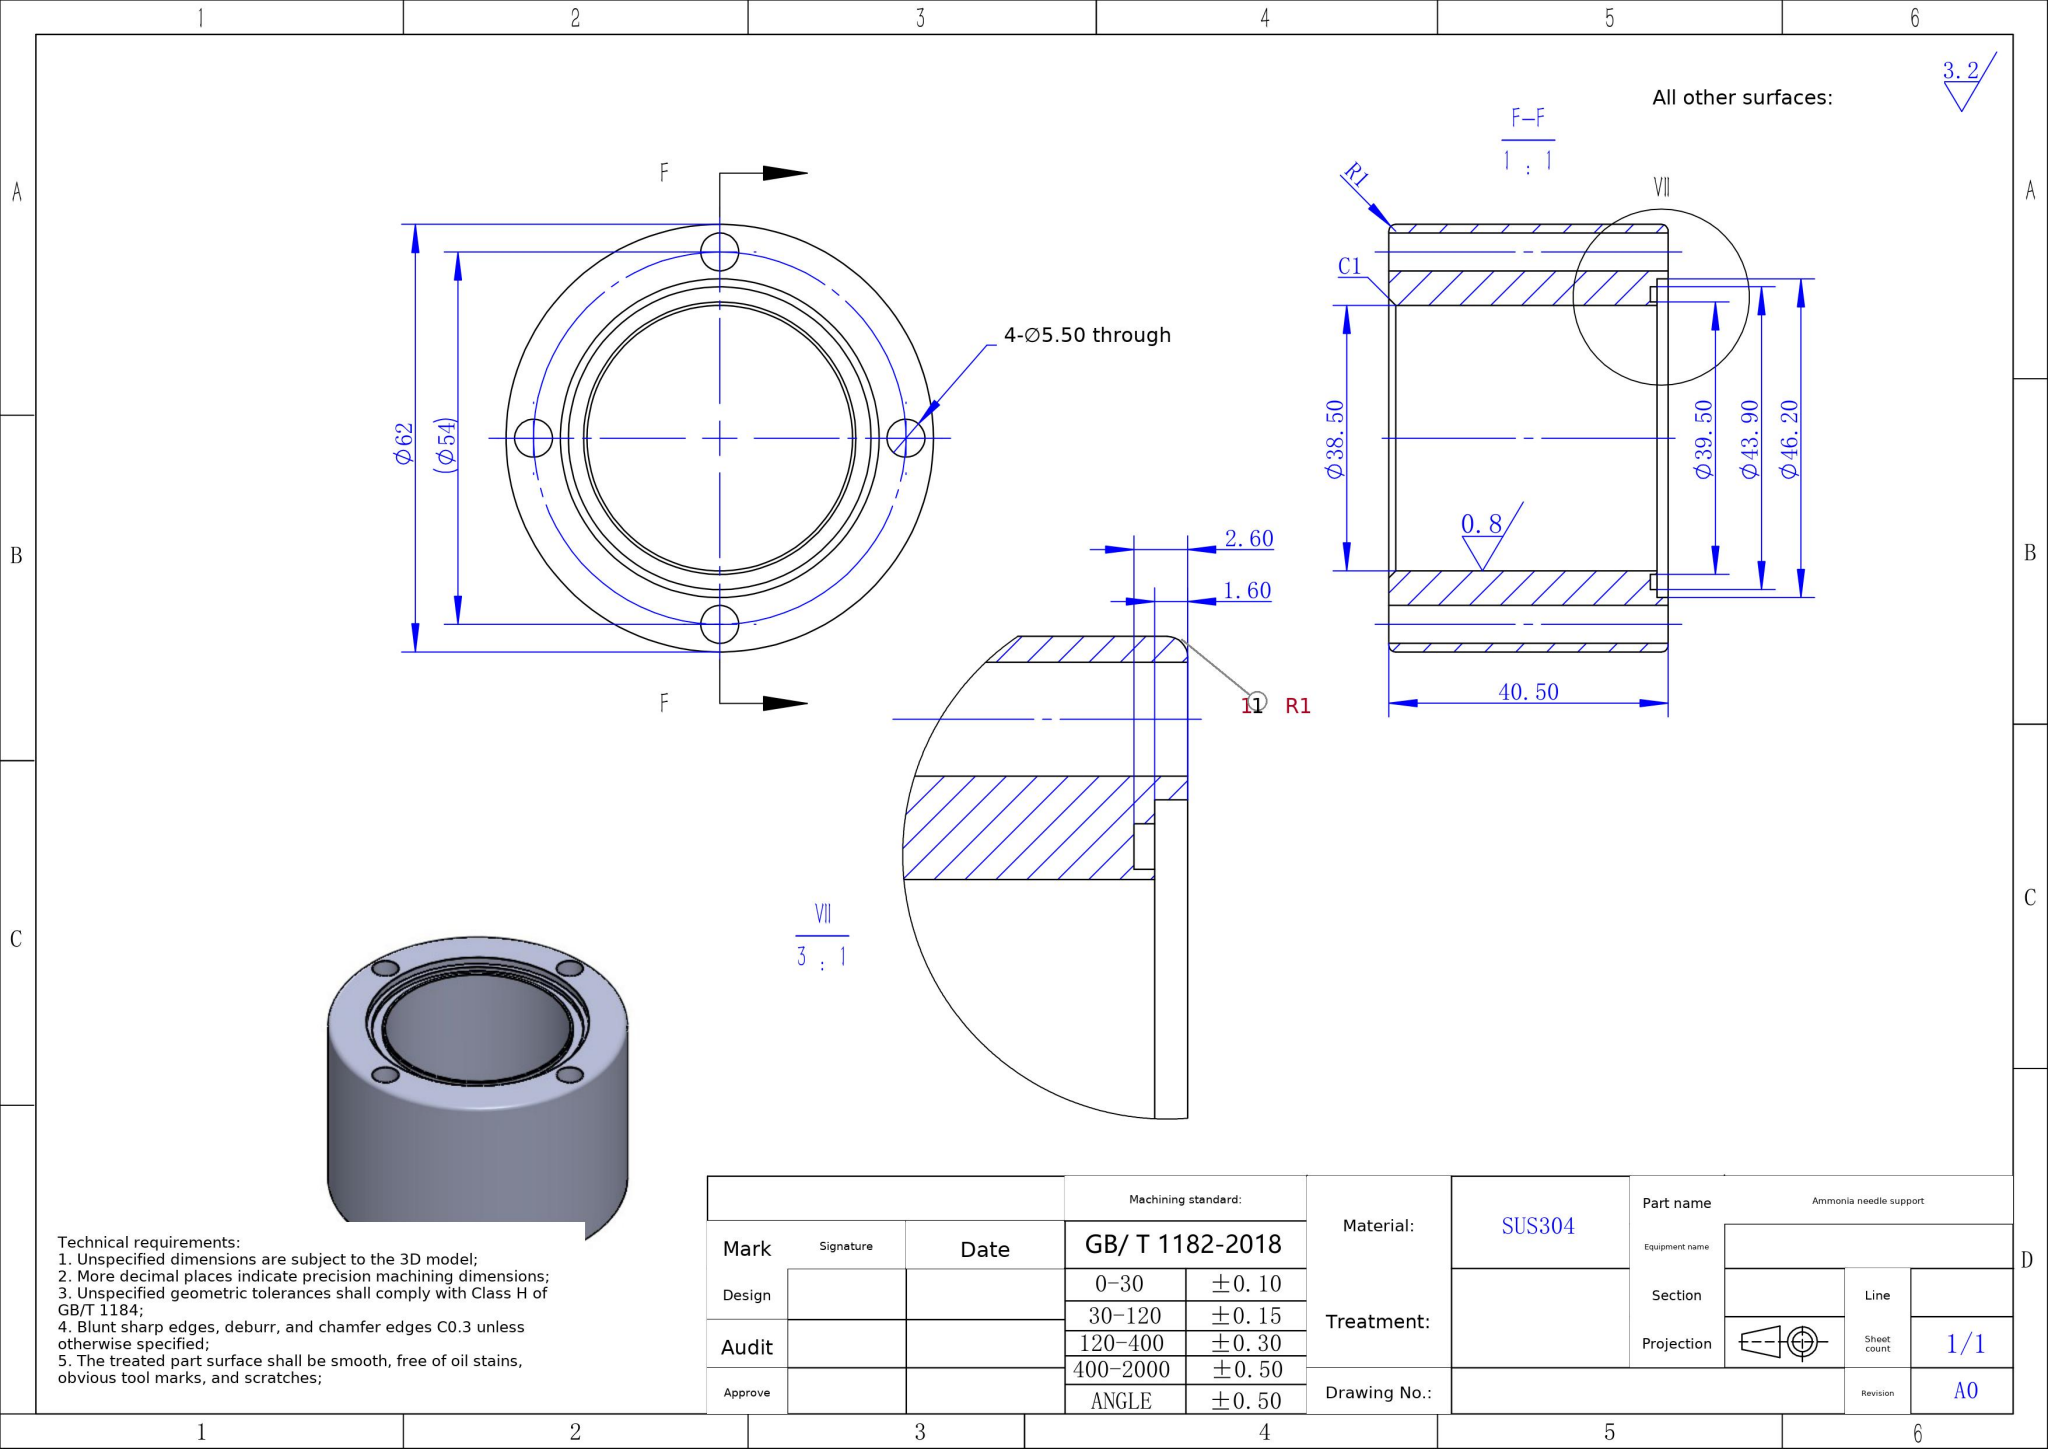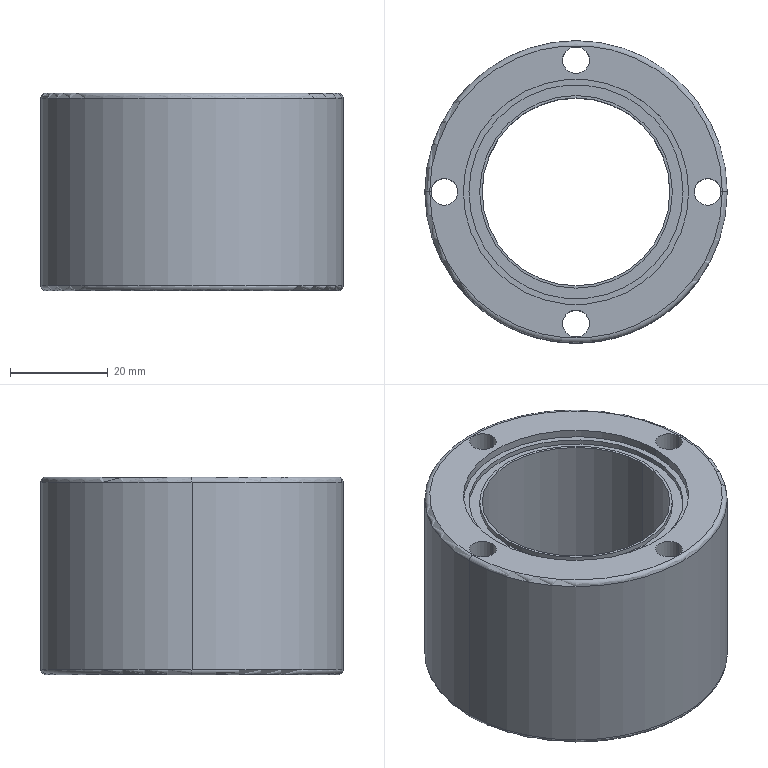Part | SolidWorks | mm | material SUS304 | 1 solid | 29 faces | box 62 x 62 x 40.5 mm | volume 70023 mm3 | cylinder 18 | plane 5 | torus 4 | cone 2 | commonest cylinder face diameters 5.5 x8 39.5 x2 43.9 x2 46.2 x2 62 x2 38.5 x2
build123d program:
from build123d import *

# Parameters (mm, degrees)
SKETCH1_R           = 31
BOSS_EXTRUDE1_DEPTH = 40.5
SKETCH2_R           = 19.25
CUT_EXTRUDE1_DEPTH  = 40.5
SKETCH3_R           = 2.75
CUT_EXTRUDE2_DEPTH  = 60.685
FILLET1_R           = 1
CHAMFER1_SIZE       = 1
SKETCH4_R           = 23.1
CUT_EXTRUDE3_DEPTH  = 1.6
SKETCH5_R           = 21.95
CUT_EXTRUDE4_DEPTH  = 1
BOSS_EXTRUDE2_START = 1
SKETCH6_R           = 19.75
SKETCH6_R_2         = 19.25
BOSS_EXTRUDE2_DEPTH = 1


with BuildPart() as part:
    # Sketch1 → Boss-Extrude1 (new body)
    with BuildSketch(Plane.XY):
        Circle(SKETCH1_R)
    extrude(amount=BOSS_EXTRUDE1_DEPTH)

    # Sketch2 → Cut-Extrude1 (cut)
    with BuildSketch(Plane.XY.offset(40.5)):
        Circle(SKETCH2_R)
    extrude(amount=-CUT_EXTRUDE1_DEPTH, mode=Mode.SUBTRACT)

    # Sketch3 → Cut-Extrude2 (cut, through all)
    with BuildSketch(Plane.XY.offset(40.5)):
        with Locations((0, 27)):
            Circle(SKETCH3_R)
        with Locations((27, 0)):
            Circle(SKETCH3_R)
        with Locations((0, -27)):
            Circle(SKETCH3_R)
        with Locations((-27, 0)):
            Circle(SKETCH3_R)
    extrude(amount=-CUT_EXTRUDE2_DEPTH, mode=Mode.SUBTRACT)

    # Fillet1
    fillet1_edges = [part.edges().sort_by_distance(p)[0] for p in [
        (-31, 0, 0),
        (-31, 0, 40.5),
    ]]
    fillet(fillet1_edges, radius=FILLET1_R)

    # Chamfer1
    chamfer1_edges = [part.edges().sort_by_distance(p)[0] for p in [
        (-19.25, 0, 0),
    ]]
    chamfer(chamfer1_edges, length=CHAMFER1_SIZE)

    # Sketch4 → Cut-Extrude3 (cut)
    with BuildSketch(Plane.XY.offset(40.5)):
        Circle(SKETCH4_R)
    extrude(amount=-CUT_EXTRUDE3_DEPTH, mode=Mode.SUBTRACT)

    # Sketch5 → Cut-Extrude4 (cut)
    with BuildSketch(Plane.XY.offset(38.9)):
        Circle(SKETCH5_R)
    extrude(amount=-CUT_EXTRUDE4_DEPTH, mode=Mode.SUBTRACT)

    # Sketch6 → Boss-Extrude2 (add)
    with BuildSketch(Plane.XY.offset(37.9).offset(BOSS_EXTRUDE2_START)):
        Circle(SKETCH6_R)
        Circle(SKETCH6_R_2, mode=Mode.SUBTRACT)
    extrude(amount=-BOSS_EXTRUDE2_DEPTH)


solid = part.part
STEP:
#1=CARTESIAN_POINT('',(19.75,0.,38.9));
#2=VERTEX_POINT('',#1);
#3=CARTESIAN_POINT('',(-19.75,0.,38.9));
#4=VERTEX_POINT('',#3);
#5=CARTESIAN_POINT('',(0.,0.,38.9));
#6=DIRECTION('',(0.,0.,1.));
#7=DIRECTION('',(1.,0.,0.));
#8=AXIS2_PLACEMENT_3D('',#5,#6,#7);
#9=CIRCLE('',#8,19.75);
#10=EDGE_CURVE('',#2,#4,#9,.T.);
#11=ORIENTED_EDGE('',*,*,#10,.F.);
#12=CARTESIAN_POINT('',(19.75,0.,37.9));
#13=VERTEX_POINT('',#12);
#14=CARTESIAN_POINT('',(19.75,0.,38.9));
#15=DIRECTION('',(0.,0.,-1.));
#16=VECTOR('',#15,1000.);
#17=LINE('',#14,#16);
#18=EDGE_CURVE('',#2,#13,#17,.T.);
#19=ORIENTED_EDGE('',*,*,#18,.T.);
#20=CARTESIAN_POINT('',(-19.75,0.,37.9));
#21=VERTEX_POINT('',#20);
#22=CARTESIAN_POINT('',(0.,0.,37.9));
#23=DIRECTION('',(0.,0.,1.));
#24=DIRECTION('',(1.,0.,0.));
#25=AXIS2_PLACEMENT_3D('',#22,#23,#24);
#26=CIRCLE('',#25,19.75);
#27=EDGE_CURVE('',#13,#21,#26,.T.);
#28=ORIENTED_EDGE('',*,*,#27,.T.);
#29=CARTESIAN_POINT('',(-19.75,0.,38.9));
#30=DIRECTION('',(0.,0.,-1.));
#31=VECTOR('',#30,1000.);
#32=LINE('',#29,#31);
#33=EDGE_CURVE('',#4,#21,#32,.T.);
#34=ORIENTED_EDGE('',*,*,#33,.F.);
#35=EDGE_LOOP('',(#11,#19,#28,#34));
#36=FACE_OUTER_BOUND('',#35,.T.);
#37=CARTESIAN_POINT('',(0.,0.,38.9));
#38=DIRECTION('',(0.,0.,-1.));
#39=DIRECTION('',(-1.,0.,0.));
#40=AXIS2_PLACEMENT_3D('',#37,#38,#39);
#41=CYLINDRICAL_SURFACE('',#40,19.75);
#42=ADVANCED_FACE('',(#36),#41,.T.);
#43=CARTESIAN_POINT('',(-21.95,0.,37.9));
#44=VERTEX_POINT('',#43);
#45=CARTESIAN_POINT('',(21.95,0.,37.9));
#46=VERTEX_POINT('',#45);
#47=CARTESIAN_POINT('',(0.,0.,37.9));
#48=DIRECTION('',(0.,0.,1.));
#49=DIRECTION('',(1.,0.,0.));
#50=AXIS2_PLACEMENT_3D('',#47,#48,#49);
#51=CIRCLE('',#50,21.95);
#52=EDGE_CURVE('',#44,#46,#51,.T.);
#53=ORIENTED_EDGE('',*,*,#52,.F.);
#54=CARTESIAN_POINT('',(-21.95,0.,38.9));
#55=VERTEX_POINT('',#54);
#56=CARTESIAN_POINT('',(-21.95,0.,37.9));
#57=DIRECTION('',(0.,0.,1.));
#58=VECTOR('',#57,1000.);
#59=LINE('',#56,#58);
#60=EDGE_CURVE('',#44,#55,#59,.T.);
#61=ORIENTED_EDGE('',*,*,#60,.T.);
#62=CARTESIAN_POINT('',(21.95,0.,38.9));
#63=VERTEX_POINT('',#62);
#64=CARTESIAN_POINT('',(0.,0.,38.9));
#65=DIRECTION('',(0.,0.,1.));
#66=DIRECTION('',(1.,0.,0.));
#67=AXIS2_PLACEMENT_3D('',#64,#65,#66);
#68=CIRCLE('',#67,21.95);
#69=EDGE_CURVE('',#55,#63,#68,.T.);
#70=ORIENTED_EDGE('',*,*,#69,.T.);
#71=CARTESIAN_POINT('',(21.95,0.,37.9));
#72=DIRECTION('',(0.,0.,1.));
#73=VECTOR('',#72,1000.);
#74=LINE('',#71,#73);
#75=EDGE_CURVE('',#46,#63,#74,.T.);
#76=ORIENTED_EDGE('',*,*,#75,.F.);
#77=EDGE_LOOP('',(#53,#61,#70,#76));
#78=FACE_OUTER_BOUND('',#77,.T.);
#79=CARTESIAN_POINT('',(0.,0.,37.9));
#80=DIRECTION('',(0.,0.,1.));
#81=DIRECTION('',(1.,0.,0.));
#82=AXIS2_PLACEMENT_3D('',#79,#80,#81);
#83=CYLINDRICAL_SURFACE('',#82,21.95);
#84=ADVANCED_FACE('',(#78),#83,.F.);
#85=CARTESIAN_POINT('',(-23.1,0.,38.9));
#86=VERTEX_POINT('',#85);
#87=CARTESIAN_POINT('',(23.1,0.,38.9));
#88=VERTEX_POINT('',#87);
#89=CARTESIAN_POINT('',(0.,0.,38.9));
#90=DIRECTION('',(0.,0.,1.));
#91=DIRECTION('',(1.,0.,0.));
#92=AXIS2_PLACEMENT_3D('',#89,#90,#91);
#93=CIRCLE('',#92,23.1);
#94=EDGE_CURVE('',#86,#88,#93,.T.);
#95=ORIENTED_EDGE('',*,*,#94,.F.);
#96=CARTESIAN_POINT('',(-23.1,0.,40.5));
#97=VERTEX_POINT('',#96);
#98=CARTESIAN_POINT('',(-23.1,0.,38.9));
#99=DIRECTION('',(0.,0.,1.));
#100=VECTOR('',#99,1000.);
#101=LINE('',#98,#100);
#102=EDGE_CURVE('',#86,#97,#101,.T.);
#103=ORIENTED_EDGE('',*,*,#102,.T.);
#104=CARTESIAN_POINT('',(23.1,0.,40.5));
#105=VERTEX_POINT('',#104);
#106=CARTESIAN_POINT('',(0.,0.,40.5));
#107=DIRECTION('',(0.,0.,1.));
#108=DIRECTION('',(1.,0.,0.));
#109=AXIS2_PLACEMENT_3D('',#106,#107,#108);
#110=CIRCLE('',#109,23.1);
#111=EDGE_CURVE('',#97,#105,#110,.T.);
#112=ORIENTED_EDGE('',*,*,#111,.T.);
#113=CARTESIAN_POINT('',(23.1,0.,38.9));
#114=DIRECTION('',(0.,0.,1.));
#115=VECTOR('',#114,1000.);
#116=LINE('',#113,#115);
#117=EDGE_CURVE('',#88,#105,#116,.T.);
#118=ORIENTED_EDGE('',*,*,#117,.F.);
#119=EDGE_LOOP('',(#95,#103,#112,#118));
#120=FACE_OUTER_BOUND('',#119,.T.);
#121=CARTESIAN_POINT('',(0.,0.,38.9));
#122=DIRECTION('',(0.,0.,1.));
#123=DIRECTION('',(1.,0.,0.));
#124=AXIS2_PLACEMENT_3D('',#121,#122,#123);
#125=CYLINDRICAL_SURFACE('',#124,23.1);
#126=ADVANCED_FACE('',(#120),#125,.F.);
#127=CARTESIAN_POINT('',(19.25,0.,1.));
#128=VERTEX_POINT('',#127);
#129=CARTESIAN_POINT('',(-19.25,0.,1.));
#130=VERTEX_POINT('',#129);
#131=CARTESIAN_POINT('',(0.,0.,1.));
#132=DIRECTION('',(0.,0.,-1.));
#133=DIRECTION('',(1.,0.,0.));
#134=AXIS2_PLACEMENT_3D('',#131,#132,#133);
#135=CIRCLE('',#134,19.25);
#136=EDGE_CURVE('',#128,#130,#135,.T.);
#137=ORIENTED_EDGE('',*,*,#136,.F.);
#138=CARTESIAN_POINT('',(20.25,0.,0.));
#139=VERTEX_POINT('',#138);
#140=CARTESIAN_POINT('',(20.25,0.,0.));
#141=DIRECTION('',(0.7071,0.,-0.7071));
#142=VECTOR('',#141,1000.);
#143=LINE('',#140,#142);
#144=EDGE_CURVE('',#128,#139,#143,.T.);
#145=ORIENTED_EDGE('',*,*,#144,.T.);
#146=CARTESIAN_POINT('',(-20.25,0.,0.));
#147=VERTEX_POINT('',#146);
#148=CARTESIAN_POINT('',(0.,0.,0.));
#149=DIRECTION('',(0.,0.,1.));
#150=DIRECTION('',(1.,0.,0.));
#151=AXIS2_PLACEMENT_3D('',#148,#149,#150);
#152=CIRCLE('',#151,20.25);
#153=EDGE_CURVE('',#147,#139,#152,.T.);
#154=ORIENTED_EDGE('',*,*,#153,.F.);
#155=CARTESIAN_POINT('',(-20.25,0.,0.));
#156=DIRECTION('',(-0.7071,0.,-0.7071));
#157=VECTOR('',#156,1000.);
#158=LINE('',#155,#157);
#159=EDGE_CURVE('',#130,#147,#158,.T.);
#160=ORIENTED_EDGE('',*,*,#159,.F.);
#161=EDGE_LOOP('',(#137,#145,#154,#160));
#162=FACE_OUTER_BOUND('',#161,.T.);
#163=CARTESIAN_POINT('',(0.,0.,0.));
#164=DIRECTION('',(0.,0.,-1.));
#165=DIRECTION('',(-1.,0.,0.));
#166=AXIS2_PLACEMENT_3D('',#163,#164,#165);
#167=CONICAL_SURFACE('',#166,20.25,0.7854);
#168=ADVANCED_FACE('',(#162),#167,.F.);
#169=CARTESIAN_POINT('',(-31.,0.,39.5));
#170=VERTEX_POINT('',#169);
#171=CARTESIAN_POINT('',(31.,0.,39.5));
#172=VERTEX_POINT('',#171);
#173=CARTESIAN_POINT('',(0.,0.,39.5));
#174=DIRECTION('',(0.,0.,-1.));
#175=DIRECTION('',(1.,0.,0.));
#176=AXIS2_PLACEMENT_3D('',#173,#174,#175);
#177=CIRCLE('',#176,31.);
#178=EDGE_CURVE('',#170,#172,#177,.T.);
#179=ORIENTED_EDGE('',*,*,#178,.F.);
#180=CARTESIAN_POINT('',(-30.,0.,40.5));
#181=VERTEX_POINT('',#180);
#182=CARTESIAN_POINT('',(-30.,0.,39.5));
#183=DIRECTION('',(0.,1.,0.));
#184=DIRECTION('',(-1.,0.,0.));
#185=AXIS2_PLACEMENT_3D('',#182,#183,#184);
#186=CIRCLE('',#185,1.);
#187=EDGE_CURVE('',#170,#181,#186,.T.);
#188=ORIENTED_EDGE('',*,*,#187,.T.);
#189=CARTESIAN_POINT('',(30.,0.,40.5));
#190=VERTEX_POINT('',#189);
#191=CARTESIAN_POINT('',(0.,0.,40.5));
#192=DIRECTION('',(0.,0.,1.));
#193=DIRECTION('',(1.,0.,0.));
#194=AXIS2_PLACEMENT_3D('',#191,#192,#193);
#195=CIRCLE('',#194,30.);
#196=EDGE_CURVE('',#190,#181,#195,.T.);
#197=ORIENTED_EDGE('',*,*,#196,.F.);
#198=CARTESIAN_POINT('',(30.,0.,39.5));
#199=DIRECTION('',(0.,-1.,0.));
#200=DIRECTION('',(0.,0.,-1.));
#201=AXIS2_PLACEMENT_3D('',#198,#199,#200);
#202=CIRCLE('',#201,1.);
#203=EDGE_CURVE('',#172,#190,#202,.T.);
#204=ORIENTED_EDGE('',*,*,#203,.F.);
#205=EDGE_LOOP('',(#179,#188,#197,#204));
#206=FACE_OUTER_BOUND('',#205,.T.);
#207=CARTESIAN_POINT('',(0.,0.,39.5));
#208=DIRECTION('',(0.,0.,1.));
#209=DIRECTION('',(1.,0.,0.));
#210=AXIS2_PLACEMENT_3D('',#207,#208,#209);
#211=TOROIDAL_SURFACE('',#210,30.,1.);
#212=ADVANCED_FACE('',(#206),#211,.T.);
#213=CARTESIAN_POINT('',(-30.,0.,0.));
#214=VERTEX_POINT('',#213);
#215=CARTESIAN_POINT('',(30.,0.,0.));
#216=VERTEX_POINT('',#215);
#217=CARTESIAN_POINT('',(0.,0.,0.));
#218=DIRECTION('',(0.,0.,-1.));
#219=DIRECTION('',(1.,0.,0.));
#220=AXIS2_PLACEMENT_3D('',#217,#218,#219);
#221=CIRCLE('',#220,30.);
#222=EDGE_CURVE('',#214,#216,#221,.T.);
#223=ORIENTED_EDGE('',*,*,#222,.F.);
#224=CARTESIAN_POINT('',(-31.,0.,1.));
#225=VERTEX_POINT('',#224);
#226=CARTESIAN_POINT('',(-30.,0.,1.));
#227=DIRECTION('',(0.,1.,0.));
#228=DIRECTION('',(-1.,0.,0.));
#229=AXIS2_PLACEMENT_3D('',#226,#227,#228);
#230=CIRCLE('',#229,1.);
#231=EDGE_CURVE('',#214,#225,#230,.T.);
#232=ORIENTED_EDGE('',*,*,#231,.T.);
#233=CARTESIAN_POINT('',(31.,0.,1.));
#234=VERTEX_POINT('',#233);
#235=CARTESIAN_POINT('',(0.,0.,1.));
#236=DIRECTION('',(0.,0.,1.));
#237=DIRECTION('',(1.,0.,0.));
#238=AXIS2_PLACEMENT_3D('',#235,#236,#237);
#239=CIRCLE('',#238,31.);
#240=EDGE_CURVE('',#234,#225,#239,.T.);
#241=ORIENTED_EDGE('',*,*,#240,.F.);
#242=CARTESIAN_POINT('',(30.,0.,1.));
#243=DIRECTION('',(0.,-1.,0.));
#244=DIRECTION('',(0.,0.,-1.));
#245=AXIS2_PLACEMENT_3D('',#242,#243,#244);
#246=CIRCLE('',#245,1.);
#247=EDGE_CURVE('',#216,#234,#246,.T.);
#248=ORIENTED_EDGE('',*,*,#247,.F.);
#249=EDGE_LOOP('',(#223,#232,#241,#248));
#250=FACE_OUTER_BOUND('',#249,.T.);
#251=CARTESIAN_POINT('',(0.,0.,1.));
#252=DIRECTION('',(0.,0.,1.));
#253=DIRECTION('',(1.,0.,0.));
#254=AXIS2_PLACEMENT_3D('',#251,#252,#253);
#255=TOROIDAL_SURFACE('',#254,30.,1.);
#256=ADVANCED_FACE('',(#250),#255,.T.);
#257=CARTESIAN_POINT('',(-2.75,27.,0.));
#258=VERTEX_POINT('',#257);
#259=CARTESIAN_POINT('',(2.75,27.,0.));
#260=VERTEX_POINT('',#259);
#261=CARTESIAN_POINT('',(0.,27.,0.));
#262=DIRECTION('',(0.,0.,1.));
#263=DIRECTION('',(1.,0.,0.));
#264=AXIS2_PLACEMENT_3D('',#261,#262,#263);
#265=CIRCLE('',#264,2.75);
#266=EDGE_CURVE('',#258,#260,#265,.T.);
#267=ORIENTED_EDGE('',*,*,#266,.F.);
#268=CARTESIAN_POINT('',(-2.75,27.,40.5));
#269=VERTEX_POINT('',#268);
#270=CARTESIAN_POINT('',(-2.75,27.,0.));
#271=DIRECTION('',(0.,0.,1.));
#272=VECTOR('',#271,1000.);
#273=LINE('',#270,#272);
#274=EDGE_CURVE('',#258,#269,#273,.T.);
#275=ORIENTED_EDGE('',*,*,#274,.T.);
#276=CARTESIAN_POINT('',(2.75,27.,40.5));
#277=VERTEX_POINT('',#276);
#278=CARTESIAN_POINT('',(0.,27.,40.5));
#279=DIRECTION('',(0.,0.,1.));
#280=DIRECTION('',(1.,0.,0.));
#281=AXIS2_PLACEMENT_3D('',#278,#279,#280);
#282=CIRCLE('',#281,2.75);
#283=EDGE_CURVE('',#269,#277,#282,.T.);
#284=ORIENTED_EDGE('',*,*,#283,.T.);
#285=CARTESIAN_POINT('',(2.75,27.,0.));
#286=DIRECTION('',(0.,0.,1.));
#287=VECTOR('',#286,1000.);
#288=LINE('',#285,#287);
#289=EDGE_CURVE('',#260,#277,#288,.T.);
#290=ORIENTED_EDGE('',*,*,#289,.F.);
#291=EDGE_LOOP('',(#267,#275,#284,#290));
#292=FACE_OUTER_BOUND('',#291,.T.);
#293=CARTESIAN_POINT('',(0.,27.,0.));
#294=DIRECTION('',(0.,0.,1.));
#295=DIRECTION('',(1.,0.,0.));
#296=AXIS2_PLACEMENT_3D('',#293,#294,#295);
#297=CYLINDRICAL_SURFACE('',#296,2.75);
#298=ADVANCED_FACE('',(#292),#297,.F.);
#299=CARTESIAN_POINT('',(24.25,-0.,0.));
#300=VERTEX_POINT('',#299);
#301=CARTESIAN_POINT('',(29.75,-0.,0.));
#302=VERTEX_POINT('',#301);
#303=CARTESIAN_POINT('',(27.,-0.,0.));
#304=DIRECTION('',(0.,0.,1.));
#305=DIRECTION('',(1.,0.,0.));
#306=AXIS2_PLACEMENT_3D('',#303,#304,#305);
#307=CIRCLE('',#306,2.75);
#308=EDGE_CURVE('',#300,#302,#307,.T.);
#309=ORIENTED_EDGE('',*,*,#308,.F.);
#310=CARTESIAN_POINT('',(24.25,-0.,40.5));
#311=VERTEX_POINT('',#310);
#312=CARTESIAN_POINT('',(24.25,-0.,0.));
#313=DIRECTION('',(0.,0.,1.));
#314=VECTOR('',#313,1000.);
#315=LINE('',#312,#314);
#316=EDGE_CURVE('',#300,#311,#315,.T.);
#317=ORIENTED_EDGE('',*,*,#316,.T.);
#318=CARTESIAN_POINT('',(29.75,-0.,40.5));
#319=VERTEX_POINT('',#318);
#320=CARTESIAN_POINT('',(27.,-0.,40.5));
#321=DIRECTION('',(0.,0.,1.));
#322=DIRECTION('',(1.,0.,0.));
#323=AXIS2_PLACEMENT_3D('',#320,#321,#322);
#324=CIRCLE('',#323,2.75);
#325=EDGE_CURVE('',#311,#319,#324,.T.);
#326=ORIENTED_EDGE('',*,*,#325,.T.);
#327=CARTESIAN_POINT('',(29.75,-0.,0.));
#328=DIRECTION('',(0.,0.,1.));
#329=VECTOR('',#328,1000.);
#330=LINE('',#327,#329);
#331=EDGE_CURVE('',#302,#319,#330,.T.);
#332=ORIENTED_EDGE('',*,*,#331,.F.);
#333=EDGE_LOOP('',(#309,#317,#326,#332));
#334=FACE_OUTER_BOUND('',#333,.T.);
#335=CARTESIAN_POINT('',(27.,-0.,0.));
#336=DIRECTION('',(0.,0.,1.));
#337=DIRECTION('',(1.,0.,0.));
#338=AXIS2_PLACEMENT_3D('',#335,#336,#337);
#339=CYLINDRICAL_SURFACE('',#338,2.75);
#340=ADVANCED_FACE('',(#334),#339,.F.);
#341=CARTESIAN_POINT('',(-2.75,-27.,0.));
#342=VERTEX_POINT('',#341);
#343=CARTESIAN_POINT('',(2.75,-27.,0.));
#344=VERTEX_POINT('',#343);
#345=CARTESIAN_POINT('',(-0.,-27.,0.));
#346=DIRECTION('',(0.,0.,1.));
#347=DIRECTION('',(1.,0.,0.));
#348=AXIS2_PLACEMENT_3D('',#345,#346,#347);
#349=CIRCLE('',#348,2.75);
#350=EDGE_CURVE('',#342,#344,#349,.T.);
#351=ORIENTED_EDGE('',*,*,#350,.F.);
#352=CARTESIAN_POINT('',(-2.75,-27.,40.5));
#353=VERTEX_POINT('',#352);
#354=CARTESIAN_POINT('',(-2.75,-27.,0.));
#355=DIRECTION('',(0.,0.,1.));
#356=VECTOR('',#355,1000.);
#357=LINE('',#354,#356);
#358=EDGE_CURVE('',#342,#353,#357,.T.);
#359=ORIENTED_EDGE('',*,*,#358,.T.);
#360=CARTESIAN_POINT('',(2.75,-27.,40.5));
#361=VERTEX_POINT('',#360);
#362=CARTESIAN_POINT('',(-0.,-27.,40.5));
#363=DIRECTION('',(0.,0.,1.));
#364=DIRECTION('',(1.,0.,0.));
#365=AXIS2_PLACEMENT_3D('',#362,#363,#364);
#366=CIRCLE('',#365,2.75);
#367=EDGE_CURVE('',#353,#361,#366,.T.);
#368=ORIENTED_EDGE('',*,*,#367,.T.);
#369=CARTESIAN_POINT('',(2.75,-27.,0.));
#370=DIRECTION('',(0.,0.,1.));
#371=VECTOR('',#370,1000.);
#372=LINE('',#369,#371);
#373=EDGE_CURVE('',#344,#361,#372,.T.);
#374=ORIENTED_EDGE('',*,*,#373,.F.);
#375=EDGE_LOOP('',(#351,#359,#368,#374));
#376=FACE_OUTER_BOUND('',#375,.T.);
#377=CARTESIAN_POINT('',(-0.,-27.,0.));
#378=DIRECTION('',(0.,0.,1.));
#379=DIRECTION('',(1.,0.,0.));
#380=AXIS2_PLACEMENT_3D('',#377,#378,#379);
#381=CYLINDRICAL_SURFACE('',#380,2.75);
#382=ADVANCED_FACE('',(#376),#381,.F.);
#383=CARTESIAN_POINT('',(-29.75,0.,0.));
#384=VERTEX_POINT('',#383);
#385=CARTESIAN_POINT('',(-24.25,0.,0.));
#386=VERTEX_POINT('',#385);
#387=CARTESIAN_POINT('',(-27.,0.,0.));
#388=DIRECTION('',(0.,0.,1.));
#389=DIRECTION('',(1.,0.,0.));
#390=AXIS2_PLACEMENT_3D('',#387,#388,#389);
#391=CIRCLE('',#390,2.75);
#392=EDGE_CURVE('',#384,#386,#391,.T.);
#393=ORIENTED_EDGE('',*,*,#392,.F.);
#394=CARTESIAN_POINT('',(-29.75,0.,40.5));
#395=VERTEX_POINT('',#394);
#396=CARTESIAN_POINT('',(-29.75,0.,0.));
#397=DIRECTION('',(0.,0.,1.));
#398=VECTOR('',#397,1000.);
#399=LINE('',#396,#398);
#400=EDGE_CURVE('',#384,#395,#399,.T.);
#401=ORIENTED_EDGE('',*,*,#400,.T.);
#402=CARTESIAN_POINT('',(-24.25,0.,40.5));
#403=VERTEX_POINT('',#402);
#404=CARTESIAN_POINT('',(-27.,0.,40.5));
#405=DIRECTION('',(0.,0.,1.));
#406=DIRECTION('',(1.,0.,0.));
#407=AXIS2_PLACEMENT_3D('',#404,#405,#406);
#408=CIRCLE('',#407,2.75);
#409=EDGE_CURVE('',#395,#403,#408,.T.);
#410=ORIENTED_EDGE('',*,*,#409,.T.);
#411=CARTESIAN_POINT('',(-24.25,0.,0.));
#412=DIRECTION('',(0.,0.,1.));
#413=VECTOR('',#412,1000.);
#414=LINE('',#411,#413);
#415=EDGE_CURVE('',#386,#403,#414,.T.);
#416=ORIENTED_EDGE('',*,*,#415,.F.);
#417=EDGE_LOOP('',(#393,#401,#410,#416));
#418=FACE_OUTER_BOUND('',#417,.T.);
#419=CARTESIAN_POINT('',(-27.,0.,0.));
#420=DIRECTION('',(0.,0.,1.));
#421=DIRECTION('',(1.,0.,0.));
#422=AXIS2_PLACEMENT_3D('',#419,#420,#421);
#423=CYLINDRICAL_SURFACE('',#422,2.75);
#424=ADVANCED_FACE('',(#418),#423,.F.);
#425=ORIENTED_EDGE('',*,*,#178,.T.);
#426=CARTESIAN_POINT('',(31.,0.,40.5));
#427=DIRECTION('',(0.,0.,-1.));
#428=VECTOR('',#427,1000.);
#429=LINE('',#426,#428);
#430=EDGE_CURVE('',#172,#234,#429,.T.);
#431=ORIENTED_EDGE('',*,*,#430,.T.);
#432=ORIENTED_EDGE('',*,*,#240,.T.);
#433=CARTESIAN_POINT('',(-31.,0.,40.5));
#434=DIRECTION('',(0.,0.,-1.));
#435=VECTOR('',#434,1000.);
#436=LINE('',#433,#435);
#437=EDGE_CURVE('',#170,#225,#436,.T.);
#438=ORIENTED_EDGE('',*,*,#437,.F.);
#439=EDGE_LOOP('',(#425,#431,#432,#438));
#440=FACE_OUTER_BOUND('',#439,.T.);
#441=CARTESIAN_POINT('',(0.,0.,40.5));
#442=DIRECTION('',(0.,0.,-1.));
#443=DIRECTION('',(-1.,0.,0.));
#444=AXIS2_PLACEMENT_3D('',#441,#442,#443);
#445=CYLINDRICAL_SURFACE('',#444,31.);
#446=ADVANCED_FACE('',(#440),#445,.T.);
#447=ORIENTED_EDGE('',*,*,#136,.T.);
#448=CARTESIAN_POINT('',(-19.25,0.,38.9));
#449=VERTEX_POINT('',#448);
#450=CARTESIAN_POINT('',(-19.25,0.,0.));
#451=DIRECTION('',(0.,0.,1.));
#452=VECTOR('',#451,1000.);
#453=LINE('',#450,#452);
#454=EDGE_CURVE('',#130,#449,#453,.T.);
#455=ORIENTED_EDGE('',*,*,#454,.T.);
#456=CARTESIAN_POINT('',(19.25,0.,38.9));
#457=VERTEX_POINT('',#456);
#458=CARTESIAN_POINT('',(0.,0.,38.9));
#459=DIRECTION('',(0.,0.,1.));
#460=DIRECTION('',(1.,0.,0.));
#461=AXIS2_PLACEMENT_3D('',#458,#459,#460);
#462=CIRCLE('',#461,19.25);
#463=EDGE_CURVE('',#449,#457,#462,.T.);
#464=ORIENTED_EDGE('',*,*,#463,.T.);
#465=CARTESIAN_POINT('',(19.25,0.,0.));
#466=DIRECTION('',(0.,0.,1.));
#467=VECTOR('',#466,1000.);
#468=LINE('',#465,#467);
#469=EDGE_CURVE('',#128,#457,#468,.T.);
#470=ORIENTED_EDGE('',*,*,#469,.F.);
#471=EDGE_LOOP('',(#447,#455,#464,#470));
#472=FACE_OUTER_BOUND('',#471,.T.);
#473=CARTESIAN_POINT('',(0.,0.,0.));
#474=DIRECTION('',(0.,0.,1.));
#475=DIRECTION('',(1.,0.,0.));
#476=AXIS2_PLACEMENT_3D('',#473,#474,#475);
#477=CYLINDRICAL_SURFACE('',#476,19.25);
#478=ADVANCED_FACE('',(#472),#477,.F.);
#479=CARTESIAN_POINT('',(0.,0.,37.9));
#480=DIRECTION('',(0.,0.,1.));
#481=DIRECTION('',(1.,0.,0.));
#482=AXIS2_PLACEMENT_3D('',#479,#480,#481);
#483=CIRCLE('',#482,21.95);
#484=EDGE_CURVE('',#46,#44,#483,.T.);
#485=ORIENTED_EDGE('',*,*,#484,.T.);
#486=ORIENTED_EDGE('',*,*,#52,.T.);
#487=EDGE_LOOP('',(#485,#486));
#488=FACE_OUTER_BOUND('',#487,.T.);
#489=CARTESIAN_POINT('',(0.,0.,37.9));
#490=DIRECTION('',(0.,0.,1.));
#491=DIRECTION('',(1.,0.,0.));
#492=AXIS2_PLACEMENT_3D('',#489,#490,#491);
#493=CIRCLE('',#492,19.75);
#494=EDGE_CURVE('',#21,#13,#493,.T.);
#495=ORIENTED_EDGE('',*,*,#494,.F.);
#496=ORIENTED_EDGE('',*,*,#27,.F.);
#497=EDGE_LOOP('',(#495,#496));
#498=FACE_BOUND('',#497,.T.);
#499=CARTESIAN_POINT('',(0.,0.,37.9));
#500=DIRECTION('',(0.,0.,1.));
#501=DIRECTION('',(1.,0.,0.));
#502=AXIS2_PLACEMENT_3D('',#499,#500,#501);
#503=PLANE('',#502);
#504=ADVANCED_FACE('',(#488,#498),#503,.T.);
#505=ORIENTED_EDGE('',*,*,#454,.F.);
#506=CARTESIAN_POINT('',(0.,0.,1.));
#507=DIRECTION('',(0.,0.,-1.));
#508=DIRECTION('',(1.,0.,0.));
#509=AXIS2_PLACEMENT_3D('',#506,#507,#508);
#510=CIRCLE('',#509,19.25);
#511=EDGE_CURVE('',#130,#128,#510,.T.);
#512=ORIENTED_EDGE('',*,*,#511,.T.);
#513=ORIENTED_EDGE('',*,*,#469,.T.);
#514=CARTESIAN_POINT('',(0.,0.,38.9));
#515=DIRECTION('',(0.,0.,1.));
#516=DIRECTION('',(1.,0.,0.));
#517=AXIS2_PLACEMENT_3D('',#514,#515,#516);
#518=CIRCLE('',#517,19.25);
#519=EDGE_CURVE('',#457,#449,#518,.T.);
#520=ORIENTED_EDGE('',*,*,#519,.T.);
#521=EDGE_LOOP('',(#505,#512,#513,#520));
#522=FACE_OUTER_BOUND('',#521,.T.);
#523=CARTESIAN_POINT('',(0.,0.,0.));
#524=DIRECTION('',(0.,0.,1.));
#525=DIRECTION('',(1.,0.,0.));
#526=AXIS2_PLACEMENT_3D('',#523,#524,#525);
#527=CYLINDRICAL_SURFACE('',#526,19.25);
#528=ADVANCED_FACE('',(#522),#527,.F.);
#529=ORIENTED_EDGE('',*,*,#430,.F.);
#530=CARTESIAN_POINT('',(0.,0.,39.5));
#531=DIRECTION('',(0.,0.,-1.));
#532=DIRECTION('',(1.,0.,0.));
#533=AXIS2_PLACEMENT_3D('',#530,#531,#532);
#534=CIRCLE('',#533,31.);
#535=EDGE_CURVE('',#172,#170,#534,.T.);
#536=ORIENTED_EDGE('',*,*,#535,.T.);
#537=ORIENTED_EDGE('',*,*,#437,.T.);
#538=CARTESIAN_POINT('',(0.,0.,1.));
#539=DIRECTION('',(0.,0.,1.));
#540=DIRECTION('',(1.,0.,0.));
#541=AXIS2_PLACEMENT_3D('',#538,#539,#540);
#542=CIRCLE('',#541,31.);
#543=EDGE_CURVE('',#225,#234,#542,.T.);
#544=ORIENTED_EDGE('',*,*,#543,.T.);
#545=EDGE_LOOP('',(#529,#536,#537,#544));
#546=FACE_OUTER_BOUND('',#545,.T.);
#547=CARTESIAN_POINT('',(0.,0.,40.5));
#548=DIRECTION('',(0.,0.,-1.));
#549=DIRECTION('',(-1.,0.,0.));
#550=AXIS2_PLACEMENT_3D('',#547,#548,#549);
#551=CYLINDRICAL_SURFACE('',#550,31.);
#552=ADVANCED_FACE('',(#546),#551,.T.);
#553=CARTESIAN_POINT('',(0.,0.,40.5));
#554=DIRECTION('',(0.,0.,1.));
#555=DIRECTION('',(1.,0.,0.));
#556=AXIS2_PLACEMENT_3D('',#553,#554,#555);
#557=CIRCLE('',#556,23.1);
#558=EDGE_CURVE('',#105,#97,#557,.T.);
#559=ORIENTED_EDGE('',*,*,#558,.F.);
#560=ORIENTED_EDGE('',*,*,#111,.F.);
#561=EDGE_LOOP('',(#559,#560));
#562=FACE_BOUND('',#561,.T.);
#563=ORIENTED_EDGE('',*,*,#196,.T.);
#564=CARTESIAN_POINT('',(0.,0.,40.5));
#565=DIRECTION('',(0.,0.,1.));
#566=DIRECTION('',(1.,0.,0.));
#567=AXIS2_PLACEMENT_3D('',#564,#565,#566);
#568=CIRCLE('',#567,30.);
#569=EDGE_CURVE('',#181,#190,#568,.T.);
#570=ORIENTED_EDGE('',*,*,#569,.T.);
#571=EDGE_LOOP('',(#563,#570));
#572=FACE_OUTER_BOUND('',#571,.T.);
#573=CARTESIAN_POINT('',(0.,27.,40.5));
#574=DIRECTION('',(0.,0.,1.));
#575=DIRECTION('',(1.,0.,0.));
#576=AXIS2_PLACEMENT_3D('',#573,#574,#575);
#577=CIRCLE('',#576,2.75);
#578=EDGE_CURVE('',#277,#269,#577,.T.);
#579=ORIENTED_EDGE('',*,*,#578,.F.);
#580=ORIENTED_EDGE('',*,*,#283,.F.);
#581=EDGE_LOOP('',(#579,#580));
#582=FACE_BOUND('',#581,.T.);
#583=CARTESIAN_POINT('',(27.,-0.,40.5));
#584=DIRECTION('',(0.,0.,1.));
#585=DIRECTION('',(1.,0.,0.));
#586=AXIS2_PLACEMENT_3D('',#583,#584,#585);
#587=CIRCLE('',#586,2.75);
#588=EDGE_CURVE('',#319,#311,#587,.T.);
#589=ORIENTED_EDGE('',*,*,#588,.F.);
#590=ORIENTED_EDGE('',*,*,#325,.F.);
#591=EDGE_LOOP('',(#589,#590));
#592=FACE_BOUND('',#591,.T.);
#593=CARTESIAN_POINT('',(-0.,-27.,40.5));
#594=DIRECTION('',(0.,0.,1.));
#595=DIRECTION('',(1.,0.,0.));
#596=AXIS2_PLACEMENT_3D('',#593,#594,#595);
#597=CIRCLE('',#596,2.75);
#598=EDGE_CURVE('',#361,#353,#597,.T.);
#599=ORIENTED_EDGE('',*,*,#598,.F.);
#600=ORIENTED_EDGE('',*,*,#367,.F.);
#601=EDGE_LOOP('',(#599,#600));
#602=FACE_BOUND('',#601,.T.);
#603=CARTESIAN_POINT('',(-27.,0.,40.5));
#604=DIRECTION('',(0.,0.,1.));
#605=DIRECTION('',(1.,0.,0.));
#606=AXIS2_PLACEMENT_3D('',#603,#604,#605);
#607=CIRCLE('',#606,2.75);
#608=EDGE_CURVE('',#403,#395,#607,.T.);
#609=ORIENTED_EDGE('',*,*,#608,.F.);
#610=ORIENTED_EDGE('',*,*,#409,.F.);
#611=EDGE_LOOP('',(#609,#610));
#612=FACE_BOUND('',#611,.T.);
#613=CARTESIAN_POINT('',(0.,0.,40.5));
#614=DIRECTION('',(0.,0.,1.));
#615=DIRECTION('',(1.,0.,0.));
#616=AXIS2_PLACEMENT_3D('',#613,#614,#615);
#617=PLANE('',#616);
#618=ADVANCED_FACE('',(#562,#572,#582,#592,#602,#612),#617,.T.);
#619=ORIENTED_EDGE('',*,*,#153,.T.);
#620=CARTESIAN_POINT('',(0.,0.,0.));
#621=DIRECTION('',(0.,0.,1.));
#622=DIRECTION('',(1.,0.,0.));
#623=AXIS2_PLACEMENT_3D('',#620,#621,#622);
#624=CIRCLE('',#623,20.25);
#625=EDGE_CURVE('',#139,#147,#624,.T.);
#626=ORIENTED_EDGE('',*,*,#625,.T.);
#627=EDGE_LOOP('',(#619,#626));
#628=FACE_BOUND('',#627,.T.);
#629=CARTESIAN_POINT('',(0.,0.,0.));
#630=DIRECTION('',(0.,0.,-1.));
#631=DIRECTION('',(1.,0.,0.));
#632=AXIS2_PLACEMENT_3D('',#629,#630,#631);
#633=CIRCLE('',#632,30.);
#634=EDGE_CURVE('',#216,#214,#633,.T.);
#635=ORIENTED_EDGE('',*,*,#634,.T.);
#636=ORIENTED_EDGE('',*,*,#222,.T.);
#637=EDGE_LOOP('',(#635,#636));
#638=FACE_OUTER_BOUND('',#637,.T.);
#639=CARTESIAN_POINT('',(0.,27.,0.));
#640=DIRECTION('',(0.,0.,1.));
#641=DIRECTION('',(1.,0.,0.));
#642=AXIS2_PLACEMENT_3D('',#639,#640,#641);
#643=CIRCLE('',#642,2.75);
#644=EDGE_CURVE('',#260,#258,#643,.T.);
#645=ORIENTED_EDGE('',*,*,#644,.T.);
#646=ORIENTED_EDGE('',*,*,#266,.T.);
#647=EDGE_LOOP('',(#645,#646));
#648=FACE_BOUND('',#647,.T.);
#649=CARTESIAN_POINT('',(27.,-0.,0.));
#650=DIRECTION('',(0.,0.,1.));
#651=DIRECTION('',(1.,0.,0.));
#652=AXIS2_PLACEMENT_3D('',#649,#650,#651);
#653=CIRCLE('',#652,2.75);
#654=EDGE_CURVE('',#302,#300,#653,.T.);
#655=ORIENTED_EDGE('',*,*,#654,.T.);
#656=ORIENTED_EDGE('',*,*,#308,.T.);
#657=EDGE_LOOP('',(#655,#656));
#658=FACE_BOUND('',#657,.T.);
#659=CARTESIAN_POINT('',(-0.,-27.,0.));
#660=DIRECTION('',(0.,0.,1.));
#661=DIRECTION('',(1.,0.,0.));
#662=AXIS2_PLACEMENT_3D('',#659,#660,#661);
#663=CIRCLE('',#662,2.75);
#664=EDGE_CURVE('',#344,#342,#663,.T.);
#665=ORIENTED_EDGE('',*,*,#664,.T.);
#666=ORIENTED_EDGE('',*,*,#350,.T.);
#667=EDGE_LOOP('',(#665,#666));
#668=FACE_BOUND('',#667,.T.);
#669=CARTESIAN_POINT('',(-27.,0.,0.));
#670=DIRECTION('',(0.,0.,1.));
#671=DIRECTION('',(1.,0.,0.));
#672=AXIS2_PLACEMENT_3D('',#669,#670,#671);
#673=CIRCLE('',#672,2.75);
#674=EDGE_CURVE('',#386,#384,#673,.T.);
#675=ORIENTED_EDGE('',*,*,#674,.T.);
#676=ORIENTED_EDGE('',*,*,#392,.T.);
#677=EDGE_LOOP('',(#675,#676));
#678=FACE_BOUND('',#677,.T.);
#679=CARTESIAN_POINT('',(0.,0.,0.));
#680=DIRECTION('',(0.,0.,1.));
#681=DIRECTION('',(1.,0.,0.));
#682=AXIS2_PLACEMENT_3D('',#679,#680,#681);
#683=PLANE('',#682);
#684=ADVANCED_FACE('',(#628,#638,#648,#658,#668,#678),#683,.F.);
#685=ORIENTED_EDGE('',*,*,#400,.F.);
#686=ORIENTED_EDGE('',*,*,#674,.F.);
#687=ORIENTED_EDGE('',*,*,#415,.T.);
#688=ORIENTED_EDGE('',*,*,#608,.T.);
#689=EDGE_LOOP('',(#685,#686,#687,#688));
#690=FACE_OUTER_BOUND('',#689,.T.);
#691=CARTESIAN_POINT('',(-27.,0.,0.));
#692=DIRECTION('',(0.,0.,1.));
#693=DIRECTION('',(1.,0.,0.));
#694=AXIS2_PLACEMENT_3D('',#691,#692,#693);
#695=CYLINDRICAL_SURFACE('',#694,2.75);
#696=ADVANCED_FACE('',(#690),#695,.F.);
#697=ORIENTED_EDGE('',*,*,#358,.F.);
#698=ORIENTED_EDGE('',*,*,#664,.F.);
#699=ORIENTED_EDGE('',*,*,#373,.T.);
#700=ORIENTED_EDGE('',*,*,#598,.T.);
#701=EDGE_LOOP('',(#697,#698,#699,#700));
#702=FACE_OUTER_BOUND('',#701,.T.);
#703=CARTESIAN_POINT('',(-0.,-27.,0.));
#704=DIRECTION('',(0.,0.,1.));
#705=DIRECTION('',(1.,0.,0.));
#706=AXIS2_PLACEMENT_3D('',#703,#704,#705);
#707=CYLINDRICAL_SURFACE('',#706,2.75);
#708=ADVANCED_FACE('',(#702),#707,.F.);
#709=ORIENTED_EDGE('',*,*,#316,.F.);
#710=ORIENTED_EDGE('',*,*,#654,.F.);
#711=ORIENTED_EDGE('',*,*,#331,.T.);
#712=ORIENTED_EDGE('',*,*,#588,.T.);
#713=EDGE_LOOP('',(#709,#710,#711,#712));
#714=FACE_OUTER_BOUND('',#713,.T.);
#715=CARTESIAN_POINT('',(27.,-0.,0.));
#716=DIRECTION('',(0.,0.,1.));
#717=DIRECTION('',(1.,0.,0.));
#718=AXIS2_PLACEMENT_3D('',#715,#716,#717);
#719=CYLINDRICAL_SURFACE('',#718,2.75);
#720=ADVANCED_FACE('',(#714),#719,.F.);
#721=ORIENTED_EDGE('',*,*,#274,.F.);
#722=ORIENTED_EDGE('',*,*,#644,.F.);
#723=ORIENTED_EDGE('',*,*,#289,.T.);
#724=ORIENTED_EDGE('',*,*,#578,.T.);
#725=EDGE_LOOP('',(#721,#722,#723,#724));
#726=FACE_OUTER_BOUND('',#725,.T.);
#727=CARTESIAN_POINT('',(0.,27.,0.));
#728=DIRECTION('',(0.,0.,1.));
#729=DIRECTION('',(1.,0.,0.));
#730=AXIS2_PLACEMENT_3D('',#727,#728,#729);
#731=CYLINDRICAL_SURFACE('',#730,2.75);
#732=ADVANCED_FACE('',(#726),#731,.F.);
#733=ORIENTED_EDGE('',*,*,#231,.F.);
#734=ORIENTED_EDGE('',*,*,#634,.F.);
#735=ORIENTED_EDGE('',*,*,#247,.T.);
#736=ORIENTED_EDGE('',*,*,#543,.F.);
#737=EDGE_LOOP('',(#733,#734,#735,#736));
#738=FACE_OUTER_BOUND('',#737,.T.);
#739=CARTESIAN_POINT('',(0.,0.,1.));
#740=DIRECTION('',(0.,0.,1.));
#741=DIRECTION('',(1.,0.,0.));
#742=AXIS2_PLACEMENT_3D('',#739,#740,#741);
#743=TOROIDAL_SURFACE('',#742,30.,1.);
#744=ADVANCED_FACE('',(#738),#743,.T.);
#745=ORIENTED_EDGE('',*,*,#187,.F.);
#746=ORIENTED_EDGE('',*,*,#535,.F.);
#747=ORIENTED_EDGE('',*,*,#203,.T.);
#748=ORIENTED_EDGE('',*,*,#569,.F.);
#749=EDGE_LOOP('',(#745,#746,#747,#748));
#750=FACE_OUTER_BOUND('',#749,.T.);
#751=CARTESIAN_POINT('',(0.,0.,39.5));
#752=DIRECTION('',(0.,0.,1.));
#753=DIRECTION('',(1.,0.,0.));
#754=AXIS2_PLACEMENT_3D('',#751,#752,#753);
#755=TOROIDAL_SURFACE('',#754,30.,1.);
#756=ADVANCED_FACE('',(#750),#755,.T.);
#757=ORIENTED_EDGE('',*,*,#144,.F.);
#758=ORIENTED_EDGE('',*,*,#511,.F.);
#759=ORIENTED_EDGE('',*,*,#159,.T.);
#760=ORIENTED_EDGE('',*,*,#625,.F.);
#761=EDGE_LOOP('',(#757,#758,#759,#760));
#762=FACE_OUTER_BOUND('',#761,.T.);
#763=CARTESIAN_POINT('',(0.,0.,0.));
#764=DIRECTION('',(0.,0.,-1.));
#765=DIRECTION('',(-1.,0.,0.));
#766=AXIS2_PLACEMENT_3D('',#763,#764,#765);
#767=CONICAL_SURFACE('',#766,20.25,0.7854);
#768=ADVANCED_FACE('',(#762),#767,.F.);
#769=CARTESIAN_POINT('',(0.,0.,38.9));
#770=DIRECTION('',(0.,0.,1.));
#771=DIRECTION('',(1.,0.,0.));
#772=AXIS2_PLACEMENT_3D('',#769,#770,#771);
#773=CIRCLE('',#772,21.95);
#774=EDGE_CURVE('',#63,#55,#773,.T.);
#775=ORIENTED_EDGE('',*,*,#774,.F.);
#776=ORIENTED_EDGE('',*,*,#69,.F.);
#777=EDGE_LOOP('',(#775,#776));
#778=FACE_BOUND('',#777,.T.);
#779=CARTESIAN_POINT('',(0.,0.,38.9));
#780=DIRECTION('',(0.,0.,1.));
#781=DIRECTION('',(1.,0.,0.));
#782=AXIS2_PLACEMENT_3D('',#779,#780,#781);
#783=CIRCLE('',#782,23.1);
#784=EDGE_CURVE('',#88,#86,#783,.T.);
#785=ORIENTED_EDGE('',*,*,#784,.T.);
#786=ORIENTED_EDGE('',*,*,#94,.T.);
#787=EDGE_LOOP('',(#785,#786));
#788=FACE_OUTER_BOUND('',#787,.T.);
#789=CARTESIAN_POINT('',(0.,0.,38.9));
#790=DIRECTION('',(0.,0.,1.));
#791=DIRECTION('',(1.,0.,0.));
#792=AXIS2_PLACEMENT_3D('',#789,#790,#791);
#793=PLANE('',#792);
#794=ADVANCED_FACE('',(#778,#788),#793,.T.);
#795=ORIENTED_EDGE('',*,*,#102,.F.);
#796=ORIENTED_EDGE('',*,*,#784,.F.);
#797=ORIENTED_EDGE('',*,*,#117,.T.);
#798=ORIENTED_EDGE('',*,*,#558,.T.);
#799=EDGE_LOOP('',(#795,#796,#797,#798));
#800=FACE_OUTER_BOUND('',#799,.T.);
#801=CARTESIAN_POINT('',(0.,0.,38.9));
#802=DIRECTION('',(0.,0.,1.));
#803=DIRECTION('',(1.,0.,0.));
#804=AXIS2_PLACEMENT_3D('',#801,#802,#803);
#805=CYLINDRICAL_SURFACE('',#804,23.1);
#806=ADVANCED_FACE('',(#800),#805,.F.);
#807=ORIENTED_EDGE('',*,*,#60,.F.);
#808=ORIENTED_EDGE('',*,*,#484,.F.);
#809=ORIENTED_EDGE('',*,*,#75,.T.);
#810=ORIENTED_EDGE('',*,*,#774,.T.);
#811=EDGE_LOOP('',(#807,#808,#809,#810));
#812=FACE_OUTER_BOUND('',#811,.T.);
#813=CARTESIAN_POINT('',(0.,0.,37.9));
#814=DIRECTION('',(0.,0.,1.));
#815=DIRECTION('',(1.,0.,0.));
#816=AXIS2_PLACEMENT_3D('',#813,#814,#815);
#817=CYLINDRICAL_SURFACE('',#816,21.95);
#818=ADVANCED_FACE('',(#812),#817,.F.);
#819=CARTESIAN_POINT('',(0.,0.,38.9));
#820=DIRECTION('',(0.,0.,1.));
#821=DIRECTION('',(1.,0.,0.));
#822=AXIS2_PLACEMENT_3D('',#819,#820,#821);
#823=CIRCLE('',#822,19.75);
#824=EDGE_CURVE('',#4,#2,#823,.T.);
#825=ORIENTED_EDGE('',*,*,#824,.T.);
#826=ORIENTED_EDGE('',*,*,#10,.T.);
#827=EDGE_LOOP('',(#825,#826));
#828=FACE_OUTER_BOUND('',#827,.T.);
#829=ORIENTED_EDGE('',*,*,#519,.F.);
#830=ORIENTED_EDGE('',*,*,#463,.F.);
#831=EDGE_LOOP('',(#829,#830));
#832=FACE_BOUND('',#831,.T.);
#833=CARTESIAN_POINT('',(0.,0.,38.9));
#834=DIRECTION('',(0.,0.,1.));
#835=DIRECTION('',(1.,0.,0.));
#836=AXIS2_PLACEMENT_3D('',#833,#834,#835);
#837=PLANE('',#836);
#838=ADVANCED_FACE('',(#828,#832),#837,.T.);
#839=ORIENTED_EDGE('',*,*,#18,.F.);
#840=ORIENTED_EDGE('',*,*,#824,.F.);
#841=ORIENTED_EDGE('',*,*,#33,.T.);
#842=ORIENTED_EDGE('',*,*,#494,.T.);
#843=EDGE_LOOP('',(#839,#840,#841,#842));
#844=FACE_OUTER_BOUND('',#843,.T.);
#845=CARTESIAN_POINT('',(0.,0.,38.9));
#846=DIRECTION('',(0.,0.,-1.));
#847=DIRECTION('',(-1.,0.,0.));
#848=AXIS2_PLACEMENT_3D('',#845,#846,#847);
#849=CYLINDRICAL_SURFACE('',#848,19.75);
#850=ADVANCED_FACE('',(#844),#849,.T.);
#851=CLOSED_SHELL('',(#42,#84,#126,#168,#212,#256,#298,#340,#382,#424,#446,#478,#504,#528,#552,#618,#684,#696,#708,#720,#732,#744,#756,#768,#794,#806,#818,#838,#850));
#852=MANIFOLD_SOLID_BREP('',#851);
#853=CARTESIAN_POINT('',(0.,0.,0.));
#854=DIRECTION('',(0.,0.,1.));
#855=DIRECTION('',(1.,0.,0.));
#856=AXIS2_PLACEMENT_3D('',#853,#854,#855);
#857=(LENGTH_UNIT()NAMED_UNIT(*)SI_UNIT(.MILLI.,.METRE.));
#858=UNCERTAINTY_MEASURE_WITH_UNIT(LENGTH_MEASURE(0.00001),#857,'','');
#859=(NAMED_UNIT(*)PLANE_ANGLE_UNIT()SI_UNIT($,.RADIAN.));
#860=(NAMED_UNIT(*)SI_UNIT($,.STERADIAN.)SOLID_ANGLE_UNIT());
#861=(GEOMETRIC_REPRESENTATION_CONTEXT(3)GLOBAL_UNCERTAINTY_ASSIGNED_CONTEXT((#858))GLOBAL_UNIT_ASSIGNED_CONTEXT((#857,#859,#860))REPRESENTATION_CONTEXT('',''));
#862=ADVANCED_BREP_SHAPE_REPRESENTATION('',(#852,#856),#861);